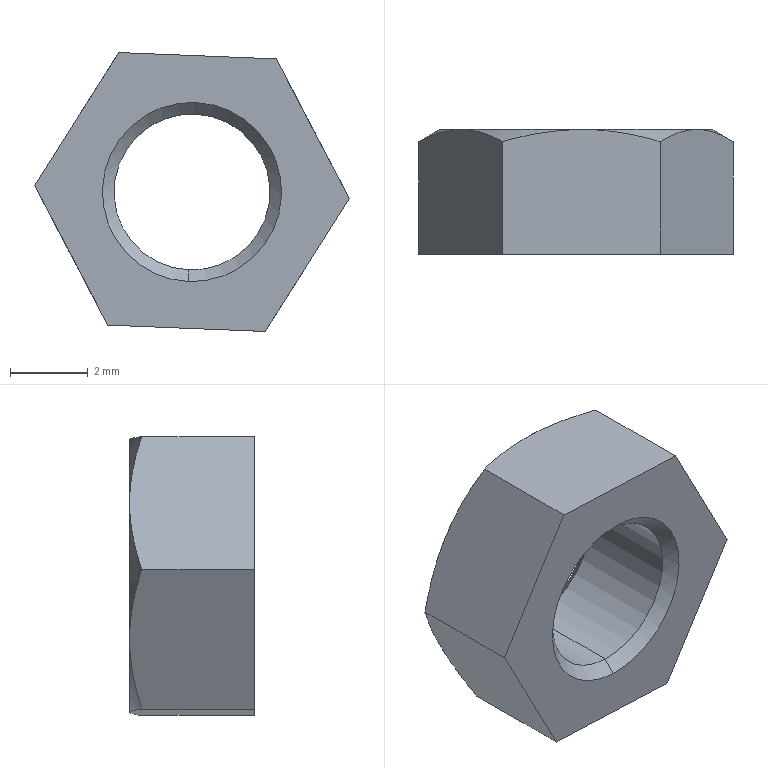Component | SolidWorks | TBK51-M4-1 | 1 solid | 20 faces | box 8.08 x 3.2 x 7.16 mm | volume 94 mm3 | cone 10 | plane 8 | cylinder 2 | commonest cylinder face diameters 4 x2
STEP:
#1=COLOUR_RGB('',0.7922,0.8196,0.9333);
#2=FILL_AREA_STYLE_COLOUR('',#1);
#3=FILL_AREA_STYLE('',(#2));
#4=SURFACE_STYLE_FILL_AREA(#3);
#5=SURFACE_SIDE_STYLE('',(#4));
#6=SURFACE_STYLE_USAGE(.BOTH.,#5);
#7=PRESENTATION_STYLE_ASSIGNMENT((#6));
#8=CARTESIAN_POINT('',(-7.38,3.112,8.653));
#9=VERTEX_POINT('',#8);
#10=CARTESIAN_POINT('',(-7.387,3.112,8.496));
#11=VERTEX_POINT('',#10);
#12=CARTESIAN_POINT('',(-7.383,3.112,8.574));
#13=DIRECTION('',(-0.,1.,0.));
#14=DIRECTION('',(-0.04067,0.,-0.9992));
#15=AXIS2_PLACEMENT_3D('',#12,#13,#14);
#16=CIRCLE('',#15,0.07874);
#17=EDGE_CURVE('',#9,#11,#16,.T.);
#18=ORIENTED_EDGE('',*,*,#17,.T.);
#19=CARTESIAN_POINT('',(-7.387,3.1,8.484));
#20=VERTEX_POINT('',#19);
#21=CARTESIAN_POINT('',(-7.387,3.112,8.496));
#22=DIRECTION('',(-0.02876,-0.7071,-0.7065));
#23=VECTOR('',#22,39.37);
#24=LINE('',#21,#23);
#25=EDGE_CURVE('',#11,#20,#24,.T.);
#26=ORIENTED_EDGE('',*,*,#25,.T.);
#27=CARTESIAN_POINT('',(-7.38,3.1,8.665));
#28=VERTEX_POINT('',#27);
#29=CARTESIAN_POINT('',(-7.383,3.1,8.574));
#30=DIRECTION('',(-0.,1.,0.));
#31=DIRECTION('',(-0.04067,0.,-0.9992));
#32=AXIS2_PLACEMENT_3D('',#29,#30,#31);
#33=CIRCLE('',#32,0.09055);
#34=EDGE_CURVE('',#28,#20,#33,.T.);
#35=ORIENTED_EDGE('',*,*,#34,.F.);
#36=CARTESIAN_POINT('',(-7.38,3.112,8.653));
#37=DIRECTION('',(0.02876,-0.7071,0.7065));
#38=VECTOR('',#37,39.37);
#39=LINE('',#36,#38);
#40=EDGE_CURVE('',#9,#28,#39,.T.);
#41=ORIENTED_EDGE('',*,*,#40,.F.);
#42=EDGE_LOOP('',(#18,#26,#35,#41));
#43=FACE_OUTER_BOUND('',#42,.T.);
#44=CARTESIAN_POINT('',(-7.383,3.112,8.574));
#45=DIRECTION('',(0.,-1.,-0.));
#46=DIRECTION('',(0.04067,0.,0.9992));
#47=AXIS2_PLACEMENT_3D('',#44,#45,#46);
#48=CONICAL_SURFACE('',#47,0.07874,0.7854);
#49=ADVANCED_FACE('',(#43),#48,.F.);
#50=ORIENTED_EDGE('',*,*,#17,.F.);
#51=CARTESIAN_POINT('',(-7.38,3.215,8.653));
#52=VERTEX_POINT('',#51);
#53=CARTESIAN_POINT('',(-7.38,1.258,8.653));
#54=DIRECTION('',(-0.,1.,0.));
#55=VECTOR('',#54,39.37);
#56=LINE('',#53,#55);
#57=EDGE_CURVE('',#9,#52,#56,.T.);
#58=ORIENTED_EDGE('',*,*,#57,.T.);
#59=CARTESIAN_POINT('',(-7.387,3.215,8.496));
#60=VERTEX_POINT('',#59);
#61=CARTESIAN_POINT('',(-7.383,3.215,8.574));
#62=DIRECTION('',(-0.,1.,0.));
#63=DIRECTION('',(-0.04067,0.,-0.9992));
#64=AXIS2_PLACEMENT_3D('',#61,#62,#63);
#65=CIRCLE('',#64,0.07874);
#66=EDGE_CURVE('',#52,#60,#65,.T.);
#67=ORIENTED_EDGE('',*,*,#66,.T.);
#68=CARTESIAN_POINT('',(-7.387,1.258,8.496));
#69=DIRECTION('',(-0.,1.,0.));
#70=VECTOR('',#69,39.37);
#71=LINE('',#68,#70);
#72=EDGE_CURVE('',#11,#60,#71,.T.);
#73=ORIENTED_EDGE('',*,*,#72,.F.);
#74=EDGE_LOOP('',(#50,#58,#67,#73));
#75=FACE_OUTER_BOUND('',#74,.T.);
#76=CARTESIAN_POINT('',(-7.383,1.258,8.574));
#77=DIRECTION('',(-0.,1.,0.));
#78=DIRECTION('',(-0.04067,0.,-0.9992));
#79=AXIS2_PLACEMENT_3D('',#76,#77,#78);
#80=CYLINDRICAL_SURFACE('',#79,0.07874);
#81=ADVANCED_FACE('',(#75),#80,.F.);
#82=ORIENTED_EDGE('',*,*,#66,.F.);
#83=CARTESIAN_POINT('',(-7.38,3.226,8.665));
#84=VERTEX_POINT('',#83);
#85=CARTESIAN_POINT('',(-7.38,3.226,8.665));
#86=DIRECTION('',(0.02876,0.7071,0.7065));
#87=VECTOR('',#86,39.37);
#88=LINE('',#85,#87);
#89=EDGE_CURVE('',#52,#84,#88,.T.);
#90=ORIENTED_EDGE('',*,*,#89,.T.);
#91=CARTESIAN_POINT('',(-7.387,3.226,8.484));
#92=VERTEX_POINT('',#91);
#93=CARTESIAN_POINT('',(-7.383,3.226,8.574));
#94=DIRECTION('',(-0.,1.,0.));
#95=DIRECTION('',(-0.04067,0.,-0.9992));
#96=AXIS2_PLACEMENT_3D('',#93,#94,#95);
#97=CIRCLE('',#96,0.09055);
#98=EDGE_CURVE('',#84,#92,#97,.T.);
#99=ORIENTED_EDGE('',*,*,#98,.T.);
#100=CARTESIAN_POINT('',(-7.387,3.226,8.484));
#101=DIRECTION('',(-0.02876,0.7071,-0.7065));
#102=VECTOR('',#101,39.37);
#103=LINE('',#100,#102);
#104=EDGE_CURVE('',#60,#92,#103,.T.);
#105=ORIENTED_EDGE('',*,*,#104,.F.);
#106=EDGE_LOOP('',(#82,#90,#99,#105));
#107=FACE_OUTER_BOUND('',#106,.T.);
#108=CARTESIAN_POINT('',(-7.383,3.226,8.574));
#109=DIRECTION('',(-0.,1.,0.));
#110=DIRECTION('',(-0.04067,0.,-0.9992));
#111=AXIS2_PLACEMENT_3D('',#108,#109,#110);
#112=CONICAL_SURFACE('',#111,0.09055,0.7854);
#113=ADVANCED_FACE('',(#107),#112,.F.);
#114=CARTESIAN_POINT('',(-7.378,3.226,8.712));
#115=VERTEX_POINT('',#114);
#116=CARTESIAN_POINT('',(-7.298,3.214,8.709));
#117=VERTEX_POINT('',#116);
#118=CARTESIAN_POINT('',(-7.378,3.226,8.712));
#119=CARTESIAN_POINT('',(-7.364,3.226,8.711));
#120=CARTESIAN_POINT('',(-7.351,3.225,8.711));
#121=CARTESIAN_POINT('',(-7.324,3.221,8.71));
#122=CARTESIAN_POINT('',(-7.311,3.218,8.709));
#123=CARTESIAN_POINT('',(-7.298,3.214,8.709));
#124=B_SPLINE_CURVE_WITH_KNOTS('',3,(#118,#119,#120,#121,#122,#123),.UNSPECIFIED.,.F.,.F.,(4,2,4),(0.01122,0.01225,0.01327),.UNSPECIFIED.);
#125=EDGE_CURVE('',#115,#117,#124,.T.);
#126=ORIENTED_EDGE('',*,*,#125,.T.);
#127=CARTESIAN_POINT('',(-7.261,3.226,8.638));
#128=VERTEX_POINT('',#127);
#129=CARTESIAN_POINT('',(-7.298,3.214,8.709));
#130=CARTESIAN_POINT('',(-7.286,3.222,8.686));
#131=CARTESIAN_POINT('',(-7.274,3.226,8.662));
#132=CARTESIAN_POINT('',(-7.261,3.226,8.638));
#133=B_SPLINE_CURVE_WITH_KNOTS('',3,(#129,#130,#131,#132),.UNSPECIFIED.,.F.,.F.,(4,4),(0.00000024,0.002045),.UNSPECIFIED.);
#134=EDGE_CURVE('',#117,#128,#133,.T.);
#135=ORIENTED_EDGE('',*,*,#134,.T.);
#136=CARTESIAN_POINT('',(-7.383,3.226,8.574));
#137=DIRECTION('',(-0.,1.,0.));
#138=DIRECTION('',(-0.04067,0.,-0.9992));
#139=AXIS2_PLACEMENT_3D('',#136,#137,#138);
#140=CIRCLE('',#139,0.1378);
#141=EDGE_CURVE('',#115,#128,#140,.T.);
#142=ORIENTED_EDGE('',*,*,#141,.F.);
#143=EDGE_LOOP('',(#126,#135,#142));
#144=FACE_OUTER_BOUND('',#143,.T.);
#145=CARTESIAN_POINT('',(-7.383,3.191,8.574));
#146=DIRECTION('',(0.,-1.,-0.));
#147=DIRECTION('',(0.04067,0.,0.9992));
#148=AXIS2_PLACEMENT_3D('',#145,#146,#147);
#149=CONICAL_SURFACE('',#148,0.1988,1.047);
#150=ADVANCED_FACE('',(#144),#149,.T.);
#151=CARTESIAN_POINT('',(-7.267,3.226,8.501));
#152=VERTEX_POINT('',#151);
#153=CARTESIAN_POINT('',(-7.383,3.226,8.574));
#154=DIRECTION('',(-0.,1.,0.));
#155=DIRECTION('',(-0.04067,0.,-0.9992));
#156=AXIS2_PLACEMENT_3D('',#153,#154,#155);
#157=CIRCLE('',#156,0.1378);
#158=EDGE_CURVE('',#128,#152,#157,.T.);
#159=ORIENTED_EDGE('',*,*,#158,.F.);
#160=CARTESIAN_POINT('',(-7.224,3.214,8.568));
#161=VERTEX_POINT('',#160);
#162=CARTESIAN_POINT('',(-7.261,3.226,8.638));
#163=CARTESIAN_POINT('',(-7.255,3.226,8.626));
#164=CARTESIAN_POINT('',(-7.249,3.225,8.614));
#165=CARTESIAN_POINT('',(-7.236,3.221,8.591));
#166=CARTESIAN_POINT('',(-7.23,3.218,8.579));
#167=CARTESIAN_POINT('',(-7.224,3.214,8.568));
#168=B_SPLINE_CURVE_WITH_KNOTS('',3,(#162,#163,#164,#165,#166,#167),.UNSPECIFIED.,.F.,.F.,(4,2,4),(0.002045,0.003063,0.004082),.UNSPECIFIED.);
#169=EDGE_CURVE('',#128,#161,#168,.T.);
#170=ORIENTED_EDGE('',*,*,#169,.T.);
#171=CARTESIAN_POINT('',(-7.224,3.214,8.568));
#172=CARTESIAN_POINT('',(-7.238,3.222,8.546));
#173=CARTESIAN_POINT('',(-7.252,3.226,8.524));
#174=CARTESIAN_POINT('',(-7.267,3.226,8.501));
#175=B_SPLINE_CURVE_WITH_KNOTS('',3,(#171,#172,#173,#174),.UNSPECIFIED.,.F.,.F.,(4,4),(0.00000024,0.002045),.UNSPECIFIED.);
#176=EDGE_CURVE('',#161,#152,#175,.T.);
#177=ORIENTED_EDGE('',*,*,#176,.T.);
#178=EDGE_LOOP('',(#159,#170,#177));
#179=FACE_OUTER_BOUND('',#178,.T.);
#180=CARTESIAN_POINT('',(-7.383,3.191,8.574));
#181=DIRECTION('',(0.,-1.,-0.));
#182=DIRECTION('',(0.04067,0.,0.9992));
#183=AXIS2_PLACEMENT_3D('',#180,#181,#182);
#184=CONICAL_SURFACE('',#183,0.1988,1.047);
#185=ADVANCED_FACE('',(#179),#184,.T.);
#186=CARTESIAN_POINT('',(-7.389,3.226,8.437));
#187=VERTEX_POINT('',#186);
#188=CARTESIAN_POINT('',(-7.383,3.226,8.574));
#189=DIRECTION('',(-0.,1.,0.));
#190=DIRECTION('',(-0.04067,0.,-0.9992));
#191=AXIS2_PLACEMENT_3D('',#188,#189,#190);
#192=CIRCLE('',#191,0.1378);
#193=EDGE_CURVE('',#152,#187,#192,.T.);
#194=ORIENTED_EDGE('',*,*,#193,.F.);
#195=CARTESIAN_POINT('',(-7.309,3.214,8.433));
#196=VERTEX_POINT('',#195);
#197=CARTESIAN_POINT('',(-7.267,3.226,8.501));
#198=CARTESIAN_POINT('',(-7.274,3.226,8.489));
#199=CARTESIAN_POINT('',(-7.281,3.225,8.478));
#200=CARTESIAN_POINT('',(-7.295,3.221,8.455));
#201=CARTESIAN_POINT('',(-7.302,3.218,8.444));
#202=CARTESIAN_POINT('',(-7.309,3.214,8.433));
#203=B_SPLINE_CURVE_WITH_KNOTS('',3,(#197,#198,#199,#200,#201,#202),.UNSPECIFIED.,.F.,.F.,(4,2,4),(0.002045,0.003063,0.004082),.UNSPECIFIED.);
#204=EDGE_CURVE('',#152,#196,#203,.T.);
#205=ORIENTED_EDGE('',*,*,#204,.T.);
#206=CARTESIAN_POINT('',(-7.309,3.214,8.433));
#207=CARTESIAN_POINT('',(-7.322,3.218,8.434));
#208=CARTESIAN_POINT('',(-7.336,3.221,8.434));
#209=CARTESIAN_POINT('',(-7.362,3.225,8.436));
#210=CARTESIAN_POINT('',(-7.375,3.226,8.436));
#211=CARTESIAN_POINT('',(-7.389,3.226,8.437));
#212=B_SPLINE_CURVE_WITH_KNOTS('',3,(#206,#207,#208,#209,#210,#211),.UNSPECIFIED.,.F.,.F.,(4,2,4),(0.003695,0.004718,0.005741),.UNSPECIFIED.);
#213=EDGE_CURVE('',#196,#187,#212,.T.);
#214=ORIENTED_EDGE('',*,*,#213,.T.);
#215=EDGE_LOOP('',(#194,#205,#214));
#216=FACE_OUTER_BOUND('',#215,.T.);
#217=CARTESIAN_POINT('',(-7.383,3.191,8.574));
#218=DIRECTION('',(0.,-1.,-0.));
#219=DIRECTION('',(0.04067,0.,0.9992));
#220=AXIS2_PLACEMENT_3D('',#217,#218,#219);
#221=CONICAL_SURFACE('',#220,0.1988,1.047);
#222=ADVANCED_FACE('',(#216),#221,.T.);
#223=CARTESIAN_POINT('',(-7.5,3.226,8.648));
#224=VERTEX_POINT('',#223);
#225=CARTESIAN_POINT('',(-7.457,3.214,8.715));
#226=VERTEX_POINT('',#225);
#227=CARTESIAN_POINT('',(-7.5,3.226,8.648));
#228=CARTESIAN_POINT('',(-7.493,3.226,8.659));
#229=CARTESIAN_POINT('',(-7.485,3.225,8.671));
#230=CARTESIAN_POINT('',(-7.471,3.221,8.693));
#231=CARTESIAN_POINT('',(-7.464,3.218,8.704));
#232=CARTESIAN_POINT('',(-7.457,3.214,8.715));
#233=B_SPLINE_CURVE_WITH_KNOTS('',3,(#227,#228,#229,#230,#231,#232),.UNSPECIFIED.,.F.,.F.,(4,2,4),(0.002045,0.003063,0.004082),.UNSPECIFIED.);
#234=EDGE_CURVE('',#224,#226,#233,.T.);
#235=ORIENTED_EDGE('',*,*,#234,.T.);
#236=CARTESIAN_POINT('',(-7.457,3.214,8.715));
#237=CARTESIAN_POINT('',(-7.444,3.218,8.715));
#238=CARTESIAN_POINT('',(-7.431,3.221,8.714));
#239=CARTESIAN_POINT('',(-7.405,3.225,8.713));
#240=CARTESIAN_POINT('',(-7.391,3.226,8.713));
#241=CARTESIAN_POINT('',(-7.378,3.226,8.712));
#242=B_SPLINE_CURVE_WITH_KNOTS('',3,(#236,#237,#238,#239,#240,#241),.UNSPECIFIED.,.F.,.F.,(4,2,4),(0.009175,0.0102,0.01122),.UNSPECIFIED.);
#243=EDGE_CURVE('',#226,#115,#242,.T.);
#244=ORIENTED_EDGE('',*,*,#243,.T.);
#245=CARTESIAN_POINT('',(-7.383,3.226,8.574));
#246=DIRECTION('',(-0.,1.,0.));
#247=DIRECTION('',(-0.04067,0.,-0.9992));
#248=AXIS2_PLACEMENT_3D('',#245,#246,#247);
#249=CIRCLE('',#248,0.1378);
#250=EDGE_CURVE('',#224,#115,#249,.T.);
#251=ORIENTED_EDGE('',*,*,#250,.F.);
#252=EDGE_LOOP('',(#235,#244,#251));
#253=FACE_OUTER_BOUND('',#252,.T.);
#254=CARTESIAN_POINT('',(-7.383,3.191,8.574));
#255=DIRECTION('',(0.,-1.,-0.));
#256=DIRECTION('',(0.04067,0.,0.9992));
#257=AXIS2_PLACEMENT_3D('',#254,#255,#256);
#258=CONICAL_SURFACE('',#257,0.1988,1.047);
#259=ADVANCED_FACE('',(#253),#258,.T.);
#260=CARTESIAN_POINT('',(-7.505,3.226,8.51));
#261=VERTEX_POINT('',#260);
#262=CARTESIAN_POINT('',(-7.383,3.226,8.574));
#263=DIRECTION('',(-0.,1.,0.));
#264=DIRECTION('',(-0.04067,0.,-0.9992));
#265=AXIS2_PLACEMENT_3D('',#262,#263,#264);
#266=CIRCLE('',#265,0.1378);
#267=EDGE_CURVE('',#187,#261,#266,.T.);
#268=ORIENTED_EDGE('',*,*,#267,.F.);
#269=CARTESIAN_POINT('',(-7.468,3.214,8.44));
#270=VERTEX_POINT('',#269);
#271=CARTESIAN_POINT('',(-7.389,3.226,8.437));
#272=CARTESIAN_POINT('',(-7.402,3.226,8.437));
#273=CARTESIAN_POINT('',(-7.416,3.225,8.438));
#274=CARTESIAN_POINT('',(-7.443,3.221,8.439));
#275=CARTESIAN_POINT('',(-7.456,3.218,8.439));
#276=CARTESIAN_POINT('',(-7.468,3.214,8.44));
#277=B_SPLINE_CURVE_WITH_KNOTS('',3,(#271,#272,#273,#274,#275,#276),.UNSPECIFIED.,.F.,.F.,(4,2,4),(0.005741,0.006764,0.007787),.UNSPECIFIED.);
#278=EDGE_CURVE('',#187,#270,#277,.T.);
#279=ORIENTED_EDGE('',*,*,#278,.T.);
#280=CARTESIAN_POINT('',(-7.468,3.214,8.44));
#281=CARTESIAN_POINT('',(-7.48,3.222,8.463));
#282=CARTESIAN_POINT('',(-7.493,3.226,8.486));
#283=CARTESIAN_POINT('',(-7.505,3.226,8.51));
#284=B_SPLINE_CURVE_WITH_KNOTS('',3,(#280,#281,#282,#283),.UNSPECIFIED.,.F.,.F.,(4,4),(0.00000024,0.002045),.UNSPECIFIED.);
#285=EDGE_CURVE('',#270,#261,#284,.T.);
#286=ORIENTED_EDGE('',*,*,#285,.T.);
#287=EDGE_LOOP('',(#268,#279,#286));
#288=FACE_OUTER_BOUND('',#287,.T.);
#289=CARTESIAN_POINT('',(-7.383,3.191,8.574));
#290=DIRECTION('',(0.,-1.,-0.));
#291=DIRECTION('',(0.04067,0.,0.9992));
#292=AXIS2_PLACEMENT_3D('',#289,#290,#291);
#293=CONICAL_SURFACE('',#292,0.1988,1.047);
#294=ADVANCED_FACE('',(#288),#293,.T.);
#295=CARTESIAN_POINT('',(-7.383,3.226,8.574));
#296=DIRECTION('',(-0.,1.,0.));
#297=DIRECTION('',(-0.04067,0.,-0.9992));
#298=AXIS2_PLACEMENT_3D('',#295,#296,#297);
#299=CIRCLE('',#298,0.09055);
#300=EDGE_CURVE('',#92,#84,#299,.T.);
#301=ORIENTED_EDGE('',*,*,#300,.F.);
#302=ORIENTED_EDGE('',*,*,#98,.F.);
#303=EDGE_LOOP('',(#301,#302));
#304=FACE_BOUND('',#303,.T.);
#305=ORIENTED_EDGE('',*,*,#267,.T.);
#306=CARTESIAN_POINT('',(-7.383,3.226,8.574));
#307=DIRECTION('',(-0.,1.,0.));
#308=DIRECTION('',(-0.04067,0.,-0.9992));
#309=AXIS2_PLACEMENT_3D('',#306,#307,#308);
#310=CIRCLE('',#309,0.1378);
#311=EDGE_CURVE('',#261,#224,#310,.T.);
#312=ORIENTED_EDGE('',*,*,#311,.T.);
#313=ORIENTED_EDGE('',*,*,#250,.T.);
#314=ORIENTED_EDGE('',*,*,#141,.T.);
#315=ORIENTED_EDGE('',*,*,#158,.T.);
#316=ORIENTED_EDGE('',*,*,#193,.T.);
#317=EDGE_LOOP('',(#305,#312,#313,#314,#315,#316));
#318=FACE_OUTER_BOUND('',#317,.T.);
#319=CARTESIAN_POINT('',(-7.521,3.226,8.58));
#320=DIRECTION('',(0.,-1.,-0.));
#321=DIRECTION('',(0.04067,-0.,0.9992));
#322=AXIS2_PLACEMENT_3D('',#319,#320,#321);
#323=PLANE('',#322);
#324=ADVANCED_FACE('',(#304,#318),#323,.F.);
#325=ORIENTED_EDGE('',*,*,#89,.F.);
#326=CARTESIAN_POINT('',(-7.383,3.215,8.574));
#327=DIRECTION('',(-0.,1.,0.));
#328=DIRECTION('',(-0.04067,0.,-0.9992));
#329=AXIS2_PLACEMENT_3D('',#326,#327,#328);
#330=CIRCLE('',#329,0.07874);
#331=EDGE_CURVE('',#60,#52,#330,.T.);
#332=ORIENTED_EDGE('',*,*,#331,.F.);
#333=ORIENTED_EDGE('',*,*,#104,.T.);
#334=ORIENTED_EDGE('',*,*,#300,.T.);
#335=EDGE_LOOP('',(#325,#332,#333,#334));
#336=FACE_OUTER_BOUND('',#335,.T.);
#337=CARTESIAN_POINT('',(-7.383,3.226,8.574));
#338=DIRECTION('',(-0.,1.,0.));
#339=DIRECTION('',(-0.04067,0.,-0.9992));
#340=AXIS2_PLACEMENT_3D('',#337,#338,#339);
#341=CONICAL_SURFACE('',#340,0.09055,0.7854);
#342=ADVANCED_FACE('',(#336),#341,.F.);
#343=ORIENTED_EDGE('',*,*,#57,.F.);
#344=CARTESIAN_POINT('',(-7.383,3.112,8.574));
#345=DIRECTION('',(-0.,1.,0.));
#346=DIRECTION('',(-0.04067,0.,-0.9992));
#347=AXIS2_PLACEMENT_3D('',#344,#345,#346);
#348=CIRCLE('',#347,0.07874);
#349=EDGE_CURVE('',#11,#9,#348,.T.);
#350=ORIENTED_EDGE('',*,*,#349,.F.);
#351=ORIENTED_EDGE('',*,*,#72,.T.);
#352=ORIENTED_EDGE('',*,*,#331,.T.);
#353=EDGE_LOOP('',(#343,#350,#351,#352));
#354=FACE_OUTER_BOUND('',#353,.T.);
#355=CARTESIAN_POINT('',(-7.383,1.258,8.574));
#356=DIRECTION('',(-0.,1.,0.));
#357=DIRECTION('',(-0.04067,0.,-0.9992));
#358=AXIS2_PLACEMENT_3D('',#355,#356,#357);
#359=CYLINDRICAL_SURFACE('',#358,0.07874);
#360=ADVANCED_FACE('',(#354),#359,.F.);
#361=ORIENTED_EDGE('',*,*,#25,.F.);
#362=ORIENTED_EDGE('',*,*,#349,.T.);
#363=ORIENTED_EDGE('',*,*,#40,.T.);
#364=CARTESIAN_POINT('',(-7.383,3.1,8.574));
#365=DIRECTION('',(-0.,1.,0.));
#366=DIRECTION('',(-0.04067,0.,-0.9992));
#367=AXIS2_PLACEMENT_3D('',#364,#365,#366);
#368=CIRCLE('',#367,0.09055);
#369=EDGE_CURVE('',#20,#28,#368,.T.);
#370=ORIENTED_EDGE('',*,*,#369,.F.);
#371=EDGE_LOOP('',(#361,#362,#363,#370));
#372=FACE_OUTER_BOUND('',#371,.T.);
#373=CARTESIAN_POINT('',(-7.383,3.112,8.574));
#374=DIRECTION('',(0.,-1.,-0.));
#375=DIRECTION('',(0.04067,0.,0.9992));
#376=AXIS2_PLACEMENT_3D('',#373,#374,#375);
#377=CONICAL_SURFACE('',#376,0.07874,0.7854);
#378=ADVANCED_FACE('',(#372),#377,.F.);
#379=CARTESIAN_POINT('',(-7.542,3.1,8.581));
#380=VERTEX_POINT('',#379);
#381=CARTESIAN_POINT('',(-7.468,3.1,8.44));
#382=VERTEX_POINT('',#381);
#383=CARTESIAN_POINT('',(-7.542,3.1,8.581));
#384=DIRECTION('',(0.4644,0.,-0.8856));
#385=VECTOR('',#384,39.37);
#386=LINE('',#383,#385);
#387=EDGE_CURVE('',#380,#382,#386,.T.);
#388=ORIENTED_EDGE('',*,*,#387,.T.);
#389=CARTESIAN_POINT('',(-7.309,3.1,8.433));
#390=VERTEX_POINT('',#389);
#391=CARTESIAN_POINT('',(-7.468,3.1,8.44));
#392=DIRECTION('',(0.9992,0.,-0.04067));
#393=VECTOR('',#392,39.37);
#394=LINE('',#391,#393);
#395=EDGE_CURVE('',#382,#390,#394,.T.);
#396=ORIENTED_EDGE('',*,*,#395,.T.);
#397=CARTESIAN_POINT('',(-7.224,3.1,8.568));
#398=VERTEX_POINT('',#397);
#399=CARTESIAN_POINT('',(-7.309,3.1,8.433));
#400=DIRECTION('',(0.5348,-0.,0.845));
#401=VECTOR('',#400,39.37);
#402=LINE('',#399,#401);
#403=EDGE_CURVE('',#390,#398,#402,.T.);
#404=ORIENTED_EDGE('',*,*,#403,.T.);
#405=CARTESIAN_POINT('',(-7.298,3.1,8.709));
#406=VERTEX_POINT('',#405);
#407=CARTESIAN_POINT('',(-7.224,3.1,8.568));
#408=DIRECTION('',(-0.4644,-0.,0.8856));
#409=VECTOR('',#408,39.37);
#410=LINE('',#407,#409);
#411=EDGE_CURVE('',#398,#406,#410,.T.);
#412=ORIENTED_EDGE('',*,*,#411,.T.);
#413=CARTESIAN_POINT('',(-7.457,3.1,8.715));
#414=VERTEX_POINT('',#413);
#415=CARTESIAN_POINT('',(-7.298,3.1,8.709));
#416=DIRECTION('',(-0.9992,-0.,0.04067));
#417=VECTOR('',#416,39.37);
#418=LINE('',#415,#417);
#419=EDGE_CURVE('',#406,#414,#418,.T.);
#420=ORIENTED_EDGE('',*,*,#419,.T.);
#421=CARTESIAN_POINT('',(-7.457,3.1,8.715));
#422=DIRECTION('',(-0.5348,0.,-0.845));
#423=VECTOR('',#422,39.37);
#424=LINE('',#421,#423);
#425=EDGE_CURVE('',#414,#380,#424,.T.);
#426=ORIENTED_EDGE('',*,*,#425,.T.);
#427=EDGE_LOOP('',(#388,#396,#404,#412,#420,#426));
#428=FACE_OUTER_BOUND('',#427,.T.);
#429=ORIENTED_EDGE('',*,*,#34,.T.);
#430=ORIENTED_EDGE('',*,*,#369,.T.);
#431=EDGE_LOOP('',(#429,#430));
#432=FACE_BOUND('',#431,.T.);
#433=CARTESIAN_POINT('',(-7.474,3.1,8.578));
#434=DIRECTION('',(-0.,1.,0.));
#435=DIRECTION('',(-0.04067,0.,-0.9992));
#436=AXIS2_PLACEMENT_3D('',#433,#434,#435);
#437=PLANE('',#436);
#438=ADVANCED_FACE('',(#428,#432),#437,.F.);
#439=CARTESIAN_POINT('',(-7.542,3.214,8.581));
#440=VERTEX_POINT('',#439);
#441=CARTESIAN_POINT('',(-7.505,3.226,8.51));
#442=CARTESIAN_POINT('',(-7.512,3.226,8.522));
#443=CARTESIAN_POINT('',(-7.518,3.225,8.534));
#444=CARTESIAN_POINT('',(-7.53,3.221,8.558));
#445=CARTESIAN_POINT('',(-7.536,3.218,8.569));
#446=CARTESIAN_POINT('',(-7.542,3.214,8.581));
#447=B_SPLINE_CURVE_WITH_KNOTS('',3,(#441,#442,#443,#444,#445,#446),.UNSPECIFIED.,.F.,.F.,(4,2,4),(0.002045,0.003063,0.004082),.UNSPECIFIED.);
#448=EDGE_CURVE('',#261,#440,#447,.T.);
#449=ORIENTED_EDGE('',*,*,#448,.T.);
#450=CARTESIAN_POINT('',(-7.542,3.214,8.581));
#451=CARTESIAN_POINT('',(-7.528,3.222,8.603));
#452=CARTESIAN_POINT('',(-7.514,3.226,8.625));
#453=CARTESIAN_POINT('',(-7.5,3.226,8.648));
#454=B_SPLINE_CURVE_WITH_KNOTS('',3,(#450,#451,#452,#453),.UNSPECIFIED.,.F.,.F.,(4,4),(0.00000024,0.002045),.UNSPECIFIED.);
#455=EDGE_CURVE('',#440,#224,#454,.T.);
#456=ORIENTED_EDGE('',*,*,#455,.T.);
#457=ORIENTED_EDGE('',*,*,#311,.F.);
#458=EDGE_LOOP('',(#449,#456,#457));
#459=FACE_OUTER_BOUND('',#458,.T.);
#460=CARTESIAN_POINT('',(-7.383,3.191,8.574));
#461=DIRECTION('',(0.,-1.,-0.));
#462=DIRECTION('',(0.04067,0.,0.9992));
#463=AXIS2_PLACEMENT_3D('',#460,#461,#462);
#464=CONICAL_SURFACE('',#463,0.1988,1.047);
#465=ADVANCED_FACE('',(#459),#464,.T.);
#466=CARTESIAN_POINT('',(-7.309,3.1,8.433));
#467=DIRECTION('',(-0.,1.,0.));
#468=VECTOR('',#467,39.37);
#469=LINE('',#466,#468);
#470=EDGE_CURVE('',#390,#196,#469,.T.);
#471=ORIENTED_EDGE('',*,*,#470,.F.);
#472=ORIENTED_EDGE('',*,*,#395,.F.);
#473=CARTESIAN_POINT('',(-7.468,3.1,8.44));
#474=DIRECTION('',(-0.,1.,0.));
#475=VECTOR('',#474,39.37);
#476=LINE('',#473,#475);
#477=EDGE_CURVE('',#382,#270,#476,.T.);
#478=ORIENTED_EDGE('',*,*,#477,.T.);
#479=ORIENTED_EDGE('',*,*,#278,.F.);
#480=ORIENTED_EDGE('',*,*,#213,.F.);
#481=EDGE_LOOP('',(#471,#472,#478,#479,#480));
#482=FACE_OUTER_BOUND('',#481,.T.);
#483=CARTESIAN_POINT('',(-7.468,3.1,8.44));
#484=DIRECTION('',(0.04067,-0.,0.9992));
#485=DIRECTION('',(-0.,1.,0.));
#486=AXIS2_PLACEMENT_3D('',#483,#484,#485);
#487=PLANE('',#486);
#488=ADVANCED_FACE('',(#482),#487,.F.);
#489=CARTESIAN_POINT('',(-7.224,3.1,8.568));
#490=DIRECTION('',(-0.,1.,0.));
#491=VECTOR('',#490,39.37);
#492=LINE('',#489,#491);
#493=EDGE_CURVE('',#398,#161,#492,.T.);
#494=ORIENTED_EDGE('',*,*,#493,.F.);
#495=ORIENTED_EDGE('',*,*,#403,.F.);
#496=ORIENTED_EDGE('',*,*,#470,.T.);
#497=ORIENTED_EDGE('',*,*,#204,.F.);
#498=ORIENTED_EDGE('',*,*,#176,.F.);
#499=EDGE_LOOP('',(#494,#495,#496,#497,#498));
#500=FACE_OUTER_BOUND('',#499,.T.);
#501=CARTESIAN_POINT('',(-7.309,3.1,8.433));
#502=DIRECTION('',(-0.845,-0.,0.5348));
#503=DIRECTION('',(-0.5348,0.,-0.845));
#504=AXIS2_PLACEMENT_3D('',#501,#502,#503);
#505=PLANE('',#504);
#506=ADVANCED_FACE('',(#500),#505,.F.);
#507=CARTESIAN_POINT('',(-7.298,3.1,8.709));
#508=DIRECTION('',(-0.,1.,0.));
#509=VECTOR('',#508,39.37);
#510=LINE('',#507,#509);
#511=EDGE_CURVE('',#406,#117,#510,.T.);
#512=ORIENTED_EDGE('',*,*,#511,.F.);
#513=ORIENTED_EDGE('',*,*,#411,.F.);
#514=ORIENTED_EDGE('',*,*,#493,.T.);
#515=ORIENTED_EDGE('',*,*,#169,.F.);
#516=ORIENTED_EDGE('',*,*,#134,.F.);
#517=EDGE_LOOP('',(#512,#513,#514,#515,#516));
#518=FACE_OUTER_BOUND('',#517,.T.);
#519=CARTESIAN_POINT('',(-7.224,3.1,8.568));
#520=DIRECTION('',(-0.8856,-0.,-0.4644));
#521=DIRECTION('',(0.4644,0.,-0.8856));
#522=AXIS2_PLACEMENT_3D('',#519,#520,#521);
#523=PLANE('',#522);
#524=ADVANCED_FACE('',(#518),#523,.F.);
#525=CARTESIAN_POINT('',(-7.457,3.1,8.715));
#526=DIRECTION('',(-0.,1.,0.));
#527=VECTOR('',#526,39.37);
#528=LINE('',#525,#527);
#529=EDGE_CURVE('',#414,#226,#528,.T.);
#530=ORIENTED_EDGE('',*,*,#529,.F.);
#531=ORIENTED_EDGE('',*,*,#419,.F.);
#532=ORIENTED_EDGE('',*,*,#511,.T.);
#533=ORIENTED_EDGE('',*,*,#125,.F.);
#534=ORIENTED_EDGE('',*,*,#243,.F.);
#535=EDGE_LOOP('',(#530,#531,#532,#533,#534));
#536=FACE_OUTER_BOUND('',#535,.T.);
#537=CARTESIAN_POINT('',(-7.298,3.1,8.709));
#538=DIRECTION('',(-0.04067,0.,-0.9992));
#539=DIRECTION('',(0.,-1.,-0.));
#540=AXIS2_PLACEMENT_3D('',#537,#538,#539);
#541=PLANE('',#540);
#542=ADVANCED_FACE('',(#536),#541,.F.);
#543=CARTESIAN_POINT('',(-7.542,3.1,8.581));
#544=DIRECTION('',(-0.,1.,0.));
#545=VECTOR('',#544,39.37);
#546=LINE('',#543,#545);
#547=EDGE_CURVE('',#380,#440,#546,.T.);
#548=ORIENTED_EDGE('',*,*,#547,.F.);
#549=ORIENTED_EDGE('',*,*,#425,.F.);
#550=ORIENTED_EDGE('',*,*,#529,.T.);
#551=ORIENTED_EDGE('',*,*,#234,.F.);
#552=ORIENTED_EDGE('',*,*,#455,.F.);
#553=EDGE_LOOP('',(#548,#549,#550,#551,#552));
#554=FACE_OUTER_BOUND('',#553,.T.);
#555=CARTESIAN_POINT('',(-7.457,3.1,8.715));
#556=DIRECTION('',(0.845,0.,-0.5348));
#557=DIRECTION('',(0.5348,-0.,0.845));
#558=AXIS2_PLACEMENT_3D('',#555,#556,#557);
#559=PLANE('',#558);
#560=ADVANCED_FACE('',(#554),#559,.F.);
#561=ORIENTED_EDGE('',*,*,#477,.F.);
#562=ORIENTED_EDGE('',*,*,#387,.F.);
#563=ORIENTED_EDGE('',*,*,#547,.T.);
#564=ORIENTED_EDGE('',*,*,#448,.F.);
#565=ORIENTED_EDGE('',*,*,#285,.F.);
#566=EDGE_LOOP('',(#561,#562,#563,#564,#565));
#567=FACE_OUTER_BOUND('',#566,.T.);
#568=CARTESIAN_POINT('',(-7.542,3.1,8.581));
#569=DIRECTION('',(0.8856,0.,0.4644));
#570=DIRECTION('',(-0.4644,-0.,0.8856));
#571=AXIS2_PLACEMENT_3D('',#568,#569,#570);
#572=PLANE('',#571);
#573=ADVANCED_FACE('',(#567),#572,.F.);
#574=CLOSED_SHELL('',(#49,#81,#113,#150,#185,#222,#259,#294,#324,#342,#360,#378,#438,#465,#488,#506,#524,#542,#560,#573));
#575=MANIFOLD_SOLID_BREP('',#574);
#576=STYLED_ITEM('',(#7),#575);
#577=(LENGTH_UNIT()NAMED_UNIT(*)SI_UNIT($,.METRE.));
#578=LENGTH_MEASURE_WITH_UNIT(LENGTH_MEASURE(0.0254),#577);
#579=DIMENSIONAL_EXPONENTS(1.,0.,0.,0.,0.,0.,0.);
#580=(CONVERSION_BASED_UNIT('',#578)LENGTH_UNIT()NAMED_UNIT(#579));
#581=UNCERTAINTY_MEASURE_WITH_UNIT(LENGTH_MEASURE(0.00001),#580,'','');
#582=(NAMED_UNIT(*)PLANE_ANGLE_UNIT()SI_UNIT($,.RADIAN.));
#583=(NAMED_UNIT(*)SI_UNIT($,.STERADIAN.)SOLID_ANGLE_UNIT());
#584=(GEOMETRIC_REPRESENTATION_CONTEXT(3)GLOBAL_UNCERTAINTY_ASSIGNED_CONTEXT((#581))GLOBAL_UNIT_ASSIGNED_CONTEXT((#580,#582,#583))REPRESENTATION_CONTEXT('',''));
#585=MECHANICAL_DESIGN_GEOMETRIC_PRESENTATION_REPRESENTATION('',(#576),#584);
#586=PRESENTATION_LAYER_ASSIGNMENT('','',(#576));
#587=CARTESIAN_POINT('',(0.,0.,0.));
#588=DIRECTION('',(0.,0.,1.));
#589=DIRECTION('',(1.,0.,0.));
#590=AXIS2_PLACEMENT_3D('',#587,#588,#589);
#591=(LENGTH_UNIT()NAMED_UNIT(*)SI_UNIT($,.METRE.));
#592=LENGTH_MEASURE_WITH_UNIT(LENGTH_MEASURE(0.0254),#591);
#593=DIMENSIONAL_EXPONENTS(1.,0.,0.,0.,0.,0.,0.);
#594=(CONVERSION_BASED_UNIT('',#592)LENGTH_UNIT()NAMED_UNIT(#593));
#595=UNCERTAINTY_MEASURE_WITH_UNIT(LENGTH_MEASURE(0.00001),#594,'','');
#596=(NAMED_UNIT(*)PLANE_ANGLE_UNIT()SI_UNIT($,.RADIAN.));
#597=(NAMED_UNIT(*)SI_UNIT($,.STERADIAN.)SOLID_ANGLE_UNIT());
#598=(GEOMETRIC_REPRESENTATION_CONTEXT(3)GLOBAL_UNCERTAINTY_ASSIGNED_CONTEXT((#595))GLOBAL_UNIT_ASSIGNED_CONTEXT((#594,#596,#597))REPRESENTATION_CONTEXT('',''));
#599=ADVANCED_BREP_SHAPE_REPRESENTATION('',(#575,#590),#598);